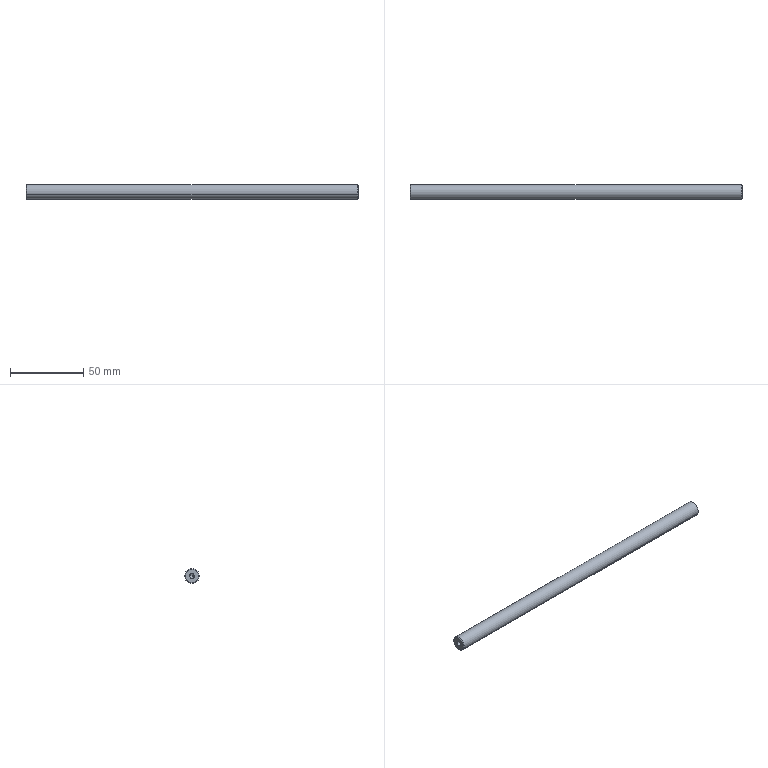Component | SolidWorks | ZL-11-14SupportRod-1 | 1 solid | 16 faces | box 226 x 10 x 10 mm | volume 17564 mm3 | cone 8 | cylinder 6 | plane 2 | commonest cylinder face diameters 3.3 x4 10 x2
build123d program:
from build123d import *

# Parameters (mm, degrees)
SKETCH1_R      = 5
EXTRUDE1_DEPTH = 113
CHAMFER1_SIZE  = 0.5


with BuildPart() as part:
    # Sketch1 → Extrude1 (new, symmetric)
    with BuildSketch(Plane(origin=(0, 0, 0), x_dir=(0, 0, -1), z_dir=(1, 0, 0))):
        Circle(SKETCH1_R)
    extrude(amount=EXTRUDE1_DEPTH, both=True)

    # Chamfer1
    chamfer1_edges = [part.edges().sort_by_distance(p)[0] for p in [
        (-113, 0, 5),
        (113, 0, 5),
    ]]
    chamfer(chamfer1_edges, length=CHAMFER1_SIZE)

    # Sketch2 → M4 Tapped Hole1 (revolve, cut)
    with BuildSketch(Plane(origin=(113, 0, 0), x_dir=(0, 0, -1), z_dir=(0, 1, 0))):
        Polygon((0, 0), (0, 11.091), (1.65, 10.1), (1.65, 0), align=None)
    m4_tapped_hole1 = revolve(axis=Axis((119.35, 0, 0), (-1, 0, 0)), mode=Mode.SUBTRACT)

    # Mirror1: M4 Tapped Hole1 across plane
    add(m4_tapped_hole1.mirror(Plane(origin=(0, 0, 0), x_dir=(0, 0, 1), z_dir=(1, 0, 0))), mode=Mode.SUBTRACT)


solid = part.part

# Placed as in the assembly
solid = solid.moved(Location((-55.448, 283.22, -56), (0, 0, 0)))
STEP:
#1=COLOUR_RGB('',0.7922,0.8196,0.9333);
#2=FILL_AREA_STYLE_COLOUR('',#1);
#3=FILL_AREA_STYLE('',(#2));
#4=SURFACE_STYLE_FILL_AREA(#3);
#5=SURFACE_SIDE_STYLE('',(#4));
#6=SURFACE_STYLE_USAGE(.BOTH.,#5);
#7=PRESENTATION_STYLE_ASSIGNMENT((#6));
#8=CARTESIAN_POINT('',(-6.195,11.15,-2.205));
#9=VERTEX_POINT('',#8);
#10=CARTESIAN_POINT('',(-6.234,11.09,-2.228));
#11=VERTEX_POINT('',#10);
#12=CARTESIAN_POINT('',(-6.234,11.09,-2.228));
#13=DIRECTION('',(-0.515,-0.8026,-0.3009));
#14=VECTOR('',#13,39.37);
#15=LINE('',#12,#14);
#16=EDGE_CURVE('',#9,#11,#15,.T.);
#17=ORIENTED_EDGE('',*,*,#16,.F.);
#18=CARTESIAN_POINT('',(-6.234,11.211,-2.182));
#19=VERTEX_POINT('',#18);
#20=CARTESIAN_POINT('',(-6.234,11.211,-2.182));
#21=DIRECTION('',(-0.515,0.8026,0.3009));
#22=VECTOR('',#21,39.37);
#23=LINE('',#20,#22);
#24=EDGE_CURVE('',#9,#19,#23,.T.);
#25=ORIENTED_EDGE('',*,*,#24,.T.);
#26=CARTESIAN_POINT('',(-6.234,11.15,-2.205));
#27=DIRECTION('',(-1.,0.,0.));
#28=DIRECTION('',(0.,-0.9364,-0.351));
#29=AXIS2_PLACEMENT_3D('',#26,#27,#28);
#30=CIRCLE('',#29,0.06496);
#31=EDGE_CURVE('',#19,#11,#30,.T.);
#32=ORIENTED_EDGE('',*,*,#31,.T.);
#33=EDGE_LOOP('',(#17,#25,#32));
#34=FACE_OUTER_BOUND('',#33,.T.);
#35=CARTESIAN_POINT('',(-6.234,11.15,-2.205));
#36=DIRECTION('',(-1.,0.,0.));
#37=DIRECTION('',(0.,-0.9364,-0.351));
#38=AXIS2_PLACEMENT_3D('',#35,#36,#37);
#39=CONICAL_SURFACE('',#38,0.06496,1.03);
#40=ADVANCED_FACE('',(#34),#39,.F.);
#41=ORIENTED_EDGE('',*,*,#31,.F.);
#42=CARTESIAN_POINT('',(-6.632,11.211,-2.182));
#43=VERTEX_POINT('',#42);
#44=CARTESIAN_POINT('',(-6.632,11.211,-2.182));
#45=DIRECTION('',(-1.,0.,0.));
#46=VECTOR('',#45,39.37);
#47=LINE('',#44,#46);
#48=EDGE_CURVE('',#19,#43,#47,.T.);
#49=ORIENTED_EDGE('',*,*,#48,.T.);
#50=CARTESIAN_POINT('',(-6.632,11.09,-2.228));
#51=VERTEX_POINT('',#50);
#52=CARTESIAN_POINT('',(-6.632,11.15,-2.205));
#53=DIRECTION('',(-1.,0.,0.));
#54=DIRECTION('',(0.,-0.9364,-0.351));
#55=AXIS2_PLACEMENT_3D('',#52,#53,#54);
#56=CIRCLE('',#55,0.06496);
#57=EDGE_CURVE('',#43,#51,#56,.T.);
#58=ORIENTED_EDGE('',*,*,#57,.T.);
#59=CARTESIAN_POINT('',(-6.632,11.09,-2.228));
#60=DIRECTION('',(-1.,0.,0.));
#61=VECTOR('',#60,39.37);
#62=LINE('',#59,#61);
#63=EDGE_CURVE('',#11,#51,#62,.T.);
#64=ORIENTED_EDGE('',*,*,#63,.F.);
#65=EDGE_LOOP('',(#41,#49,#58,#64));
#66=FACE_OUTER_BOUND('',#65,.T.);
#67=CARTESIAN_POINT('',(-6.632,11.15,-2.205));
#68=DIRECTION('',(-1.,0.,0.));
#69=DIRECTION('',(0.,-0.9364,-0.351));
#70=AXIS2_PLACEMENT_3D('',#67,#68,#69);
#71=CYLINDRICAL_SURFACE('',#70,0.06496);
#72=ADVANCED_FACE('',(#66),#71,.F.);
#73=CARTESIAN_POINT('',(1.829,11.15,-2.205));
#74=VERTEX_POINT('',#73);
#75=CARTESIAN_POINT('',(1.868,11.211,-2.182));
#76=VERTEX_POINT('',#75);
#77=CARTESIAN_POINT('',(1.868,11.211,-2.182));
#78=DIRECTION('',(0.515,0.8026,0.3009));
#79=VECTOR('',#78,39.37);
#80=LINE('',#77,#79);
#81=EDGE_CURVE('',#74,#76,#80,.T.);
#82=ORIENTED_EDGE('',*,*,#81,.F.);
#83=CARTESIAN_POINT('',(1.868,11.09,-2.228));
#84=VERTEX_POINT('',#83);
#85=CARTESIAN_POINT('',(1.868,11.09,-2.228));
#86=DIRECTION('',(0.515,-0.8026,-0.3009));
#87=VECTOR('',#86,39.37);
#88=LINE('',#85,#87);
#89=EDGE_CURVE('',#74,#84,#88,.T.);
#90=ORIENTED_EDGE('',*,*,#89,.T.);
#91=CARTESIAN_POINT('',(1.868,11.15,-2.205));
#92=DIRECTION('',(1.,0.,0.));
#93=DIRECTION('',(0.,0.9364,0.351));
#94=AXIS2_PLACEMENT_3D('',#91,#92,#93);
#95=CIRCLE('',#94,0.06496);
#96=EDGE_CURVE('',#84,#76,#95,.T.);
#97=ORIENTED_EDGE('',*,*,#96,.T.);
#98=EDGE_LOOP('',(#82,#90,#97));
#99=FACE_OUTER_BOUND('',#98,.T.);
#100=CARTESIAN_POINT('',(1.868,11.15,-2.205));
#101=DIRECTION('',(1.,0.,0.));
#102=DIRECTION('',(0.,0.9364,0.351));
#103=AXIS2_PLACEMENT_3D('',#100,#101,#102);
#104=CONICAL_SURFACE('',#103,0.06496,1.03);
#105=ADVANCED_FACE('',(#99),#104,.F.);
#106=ORIENTED_EDGE('',*,*,#96,.F.);
#107=CARTESIAN_POINT('',(2.266,11.09,-2.228));
#108=VERTEX_POINT('',#107);
#109=CARTESIAN_POINT('',(2.266,11.09,-2.228));
#110=DIRECTION('',(1.,0.,0.));
#111=VECTOR('',#110,39.37);
#112=LINE('',#109,#111);
#113=EDGE_CURVE('',#84,#108,#112,.T.);
#114=ORIENTED_EDGE('',*,*,#113,.T.);
#115=CARTESIAN_POINT('',(2.266,11.211,-2.182));
#116=VERTEX_POINT('',#115);
#117=CARTESIAN_POINT('',(2.266,11.15,-2.205));
#118=DIRECTION('',(1.,0.,0.));
#119=DIRECTION('',(0.,0.9364,0.351));
#120=AXIS2_PLACEMENT_3D('',#117,#118,#119);
#121=CIRCLE('',#120,0.06496);
#122=EDGE_CURVE('',#108,#116,#121,.T.);
#123=ORIENTED_EDGE('',*,*,#122,.T.);
#124=CARTESIAN_POINT('',(2.266,11.211,-2.182));
#125=DIRECTION('',(1.,0.,0.));
#126=VECTOR('',#125,39.37);
#127=LINE('',#124,#126);
#128=EDGE_CURVE('',#76,#116,#127,.T.);
#129=ORIENTED_EDGE('',*,*,#128,.F.);
#130=EDGE_LOOP('',(#106,#114,#123,#129));
#131=FACE_OUTER_BOUND('',#130,.T.);
#132=CARTESIAN_POINT('',(2.266,11.15,-2.205));
#133=DIRECTION('',(1.,0.,0.));
#134=DIRECTION('',(0.,0.9364,0.351));
#135=AXIS2_PLACEMENT_3D('',#132,#133,#134);
#136=CYLINDRICAL_SURFACE('',#135,0.06496);
#137=ADVANCED_FACE('',(#131),#136,.F.);
#138=CARTESIAN_POINT('',(-6.632,10.984,-2.267));
#139=VERTEX_POINT('',#138);
#140=CARTESIAN_POINT('',(-6.632,11.316,-2.143));
#141=VERTEX_POINT('',#140);
#142=CARTESIAN_POINT('',(-6.632,11.15,-2.205));
#143=DIRECTION('',(-1.,0.,0.));
#144=DIRECTION('',(0.,0.9364,0.351));
#145=AXIS2_PLACEMENT_3D('',#142,#143,#144);
#146=CIRCLE('',#145,0.1772);
#147=EDGE_CURVE('',#139,#141,#146,.T.);
#148=ORIENTED_EDGE('',*,*,#147,.F.);
#149=CARTESIAN_POINT('',(-6.612,10.966,-2.274));
#150=VERTEX_POINT('',#149);
#151=CARTESIAN_POINT('',(-6.612,10.966,-2.274));
#152=DIRECTION('',(0.7071,-0.6621,-0.2482));
#153=VECTOR('',#152,39.37);
#154=LINE('',#151,#153);
#155=EDGE_CURVE('',#139,#150,#154,.T.);
#156=ORIENTED_EDGE('',*,*,#155,.T.);
#157=CARTESIAN_POINT('',(-6.612,11.335,-2.136));
#158=VERTEX_POINT('',#157);
#159=CARTESIAN_POINT('',(-6.612,11.15,-2.205));
#160=DIRECTION('',(1.,0.,0.));
#161=DIRECTION('',(0.,0.9364,0.351));
#162=AXIS2_PLACEMENT_3D('',#159,#160,#161);
#163=CIRCLE('',#162,0.1969);
#164=EDGE_CURVE('',#158,#150,#163,.T.);
#165=ORIENTED_EDGE('',*,*,#164,.F.);
#166=CARTESIAN_POINT('',(-6.612,11.335,-2.136));
#167=DIRECTION('',(0.7071,0.6621,0.2482));
#168=VECTOR('',#167,39.37);
#169=LINE('',#166,#168);
#170=EDGE_CURVE('',#141,#158,#169,.T.);
#171=ORIENTED_EDGE('',*,*,#170,.F.);
#172=EDGE_LOOP('',(#148,#156,#165,#171));
#173=FACE_OUTER_BOUND('',#172,.T.);
#174=CARTESIAN_POINT('',(-6.612,11.15,-2.205));
#175=DIRECTION('',(1.,0.,0.));
#176=DIRECTION('',(0.,0.9364,0.351));
#177=AXIS2_PLACEMENT_3D('',#174,#175,#176);
#178=CONICAL_SURFACE('',#177,0.1969,0.7854);
#179=ADVANCED_FACE('',(#173),#178,.T.);
#180=CARTESIAN_POINT('',(2.266,11.316,-2.143));
#181=VERTEX_POINT('',#180);
#182=CARTESIAN_POINT('',(2.266,10.984,-2.267));
#183=VERTEX_POINT('',#182);
#184=CARTESIAN_POINT('',(2.266,11.15,-2.205));
#185=DIRECTION('',(1.,0.,0.));
#186=DIRECTION('',(0.,0.9364,0.351));
#187=AXIS2_PLACEMENT_3D('',#184,#185,#186);
#188=CIRCLE('',#187,0.1772);
#189=EDGE_CURVE('',#181,#183,#188,.T.);
#190=ORIENTED_EDGE('',*,*,#189,.F.);
#191=CARTESIAN_POINT('',(2.246,11.335,-2.136));
#192=VERTEX_POINT('',#191);
#193=CARTESIAN_POINT('',(2.266,11.316,-2.143));
#194=DIRECTION('',(-0.7071,0.6621,0.2482));
#195=VECTOR('',#194,39.37);
#196=LINE('',#193,#195);
#197=EDGE_CURVE('',#181,#192,#196,.T.);
#198=ORIENTED_EDGE('',*,*,#197,.T.);
#199=CARTESIAN_POINT('',(2.246,10.966,-2.274));
#200=VERTEX_POINT('',#199);
#201=CARTESIAN_POINT('',(2.246,11.15,-2.205));
#202=DIRECTION('',(-1.,0.,0.));
#203=DIRECTION('',(0.,0.9364,0.351));
#204=AXIS2_PLACEMENT_3D('',#201,#202,#203);
#205=CIRCLE('',#204,0.1969);
#206=EDGE_CURVE('',#200,#192,#205,.T.);
#207=ORIENTED_EDGE('',*,*,#206,.F.);
#208=CARTESIAN_POINT('',(2.266,10.984,-2.267));
#209=DIRECTION('',(-0.7071,-0.6621,-0.2482));
#210=VECTOR('',#209,39.37);
#211=LINE('',#208,#210);
#212=EDGE_CURVE('',#183,#200,#211,.T.);
#213=ORIENTED_EDGE('',*,*,#212,.F.);
#214=EDGE_LOOP('',(#190,#198,#207,#213));
#215=FACE_OUTER_BOUND('',#214,.T.);
#216=CARTESIAN_POINT('',(2.266,11.15,-2.205));
#217=DIRECTION('',(-1.,0.,0.));
#218=DIRECTION('',(0.,-0.9364,-0.351));
#219=AXIS2_PLACEMENT_3D('',#216,#217,#218);
#220=CONICAL_SURFACE('',#219,0.1772,0.7854);
#221=ADVANCED_FACE('',(#215),#220,.T.);
#222=ORIENTED_EDGE('',*,*,#206,.T.);
#223=CARTESIAN_POINT('',(2.266,11.335,-2.136));
#224=DIRECTION('',(-1.,0.,0.));
#225=VECTOR('',#224,39.37);
#226=LINE('',#223,#225);
#227=EDGE_CURVE('',#192,#158,#226,.T.);
#228=ORIENTED_EDGE('',*,*,#227,.T.);
#229=ORIENTED_EDGE('',*,*,#164,.T.);
#230=CARTESIAN_POINT('',(2.266,10.966,-2.274));
#231=DIRECTION('',(-1.,0.,0.));
#232=VECTOR('',#231,39.37);
#233=LINE('',#230,#232);
#234=EDGE_CURVE('',#200,#150,#233,.T.);
#235=ORIENTED_EDGE('',*,*,#234,.F.);
#236=EDGE_LOOP('',(#222,#228,#229,#235));
#237=FACE_OUTER_BOUND('',#236,.T.);
#238=CARTESIAN_POINT('',(2.266,11.15,-2.205));
#239=DIRECTION('',(-1.,0.,0.));
#240=DIRECTION('',(0.,-0.9364,-0.351));
#241=AXIS2_PLACEMENT_3D('',#238,#239,#240);
#242=CYLINDRICAL_SURFACE('',#241,0.1969);
#243=ADVANCED_FACE('',(#237),#242,.T.);
#244=ORIENTED_EDGE('',*,*,#227,.F.);
#245=CARTESIAN_POINT('',(2.246,11.15,-2.205));
#246=DIRECTION('',(-1.,0.,0.));
#247=DIRECTION('',(0.,0.9364,0.351));
#248=AXIS2_PLACEMENT_3D('',#245,#246,#247);
#249=CIRCLE('',#248,0.1969);
#250=EDGE_CURVE('',#192,#200,#249,.T.);
#251=ORIENTED_EDGE('',*,*,#250,.T.);
#252=ORIENTED_EDGE('',*,*,#234,.T.);
#253=CARTESIAN_POINT('',(-6.612,11.15,-2.205));
#254=DIRECTION('',(1.,0.,0.));
#255=DIRECTION('',(0.,0.9364,0.351));
#256=AXIS2_PLACEMENT_3D('',#253,#254,#255);
#257=CIRCLE('',#256,0.1969);
#258=EDGE_CURVE('',#150,#158,#257,.T.);
#259=ORIENTED_EDGE('',*,*,#258,.T.);
#260=EDGE_LOOP('',(#244,#251,#252,#259));
#261=FACE_OUTER_BOUND('',#260,.T.);
#262=CARTESIAN_POINT('',(2.266,11.15,-2.205));
#263=DIRECTION('',(-1.,0.,0.));
#264=DIRECTION('',(0.,-0.9364,-0.351));
#265=AXIS2_PLACEMENT_3D('',#262,#263,#264);
#266=CYLINDRICAL_SURFACE('',#265,0.1969);
#267=ADVANCED_FACE('',(#261),#266,.T.);
#268=CARTESIAN_POINT('',(2.266,11.15,-2.205));
#269=DIRECTION('',(1.,0.,0.));
#270=DIRECTION('',(0.,0.9364,0.351));
#271=AXIS2_PLACEMENT_3D('',#268,#269,#270);
#272=CIRCLE('',#271,0.06496);
#273=EDGE_CURVE('',#116,#108,#272,.T.);
#274=ORIENTED_EDGE('',*,*,#273,.F.);
#275=ORIENTED_EDGE('',*,*,#122,.F.);
#276=EDGE_LOOP('',(#274,#275));
#277=FACE_BOUND('',#276,.T.);
#278=CARTESIAN_POINT('',(2.266,11.15,-2.205));
#279=DIRECTION('',(1.,0.,0.));
#280=DIRECTION('',(0.,0.9364,0.351));
#281=AXIS2_PLACEMENT_3D('',#278,#279,#280);
#282=CIRCLE('',#281,0.1772);
#283=EDGE_CURVE('',#183,#181,#282,.T.);
#284=ORIENTED_EDGE('',*,*,#283,.T.);
#285=ORIENTED_EDGE('',*,*,#189,.T.);
#286=EDGE_LOOP('',(#284,#285));
#287=FACE_OUTER_BOUND('',#286,.T.);
#288=CARTESIAN_POINT('',(2.266,11.15,-2.205));
#289=DIRECTION('',(1.,0.,0.));
#290=DIRECTION('',(0.,0.9364,0.351));
#291=AXIS2_PLACEMENT_3D('',#288,#289,#290);
#292=PLANE('',#291);
#293=ADVANCED_FACE('',(#277,#287),#292,.T.);
#294=CARTESIAN_POINT('',(-6.632,11.15,-2.205));
#295=DIRECTION('',(-1.,0.,0.));
#296=DIRECTION('',(0.,-0.9364,-0.351));
#297=AXIS2_PLACEMENT_3D('',#294,#295,#296);
#298=CIRCLE('',#297,0.06496);
#299=EDGE_CURVE('',#51,#43,#298,.T.);
#300=ORIENTED_EDGE('',*,*,#299,.F.);
#301=ORIENTED_EDGE('',*,*,#57,.F.);
#302=EDGE_LOOP('',(#300,#301));
#303=FACE_BOUND('',#302,.T.);
#304=CARTESIAN_POINT('',(-6.632,11.15,-2.205));
#305=DIRECTION('',(-1.,0.,0.));
#306=DIRECTION('',(0.,0.9364,0.351));
#307=AXIS2_PLACEMENT_3D('',#304,#305,#306);
#308=CIRCLE('',#307,0.1772);
#309=EDGE_CURVE('',#141,#139,#308,.T.);
#310=ORIENTED_EDGE('',*,*,#309,.T.);
#311=ORIENTED_EDGE('',*,*,#147,.T.);
#312=EDGE_LOOP('',(#310,#311));
#313=FACE_OUTER_BOUND('',#312,.T.);
#314=CARTESIAN_POINT('',(-6.632,11.15,-2.205));
#315=DIRECTION('',(1.,0.,0.));
#316=DIRECTION('',(0.,0.9364,0.351));
#317=AXIS2_PLACEMENT_3D('',#314,#315,#316);
#318=PLANE('',#317);
#319=ADVANCED_FACE('',(#303,#313),#318,.F.);
#320=ORIENTED_EDGE('',*,*,#197,.F.);
#321=ORIENTED_EDGE('',*,*,#283,.F.);
#322=ORIENTED_EDGE('',*,*,#212,.T.);
#323=ORIENTED_EDGE('',*,*,#250,.F.);
#324=EDGE_LOOP('',(#320,#321,#322,#323));
#325=FACE_OUTER_BOUND('',#324,.T.);
#326=CARTESIAN_POINT('',(2.266,11.15,-2.205));
#327=DIRECTION('',(-1.,0.,0.));
#328=DIRECTION('',(0.,-0.9364,-0.351));
#329=AXIS2_PLACEMENT_3D('',#326,#327,#328);
#330=CONICAL_SURFACE('',#329,0.1772,0.7854);
#331=ADVANCED_FACE('',(#325),#330,.T.);
#332=ORIENTED_EDGE('',*,*,#155,.F.);
#333=ORIENTED_EDGE('',*,*,#309,.F.);
#334=ORIENTED_EDGE('',*,*,#170,.T.);
#335=ORIENTED_EDGE('',*,*,#258,.F.);
#336=EDGE_LOOP('',(#332,#333,#334,#335));
#337=FACE_OUTER_BOUND('',#336,.T.);
#338=CARTESIAN_POINT('',(-6.612,11.15,-2.205));
#339=DIRECTION('',(1.,0.,0.));
#340=DIRECTION('',(0.,0.9364,0.351));
#341=AXIS2_PLACEMENT_3D('',#338,#339,#340);
#342=CONICAL_SURFACE('',#341,0.1969,0.7854);
#343=ADVANCED_FACE('',(#337),#342,.T.);
#344=ORIENTED_EDGE('',*,*,#113,.F.);
#345=CARTESIAN_POINT('',(1.868,11.15,-2.205));
#346=DIRECTION('',(1.,0.,0.));
#347=DIRECTION('',(0.,0.9364,0.351));
#348=AXIS2_PLACEMENT_3D('',#345,#346,#347);
#349=CIRCLE('',#348,0.06496);
#350=EDGE_CURVE('',#76,#84,#349,.T.);
#351=ORIENTED_EDGE('',*,*,#350,.F.);
#352=ORIENTED_EDGE('',*,*,#128,.T.);
#353=ORIENTED_EDGE('',*,*,#273,.T.);
#354=EDGE_LOOP('',(#344,#351,#352,#353));
#355=FACE_OUTER_BOUND('',#354,.T.);
#356=CARTESIAN_POINT('',(2.266,11.15,-2.205));
#357=DIRECTION('',(1.,0.,0.));
#358=DIRECTION('',(0.,0.9364,0.351));
#359=AXIS2_PLACEMENT_3D('',#356,#357,#358);
#360=CYLINDRICAL_SURFACE('',#359,0.06496);
#361=ADVANCED_FACE('',(#355),#360,.F.);
#362=ORIENTED_EDGE('',*,*,#89,.F.);
#363=ORIENTED_EDGE('',*,*,#81,.T.);
#364=ORIENTED_EDGE('',*,*,#350,.T.);
#365=EDGE_LOOP('',(#362,#363,#364));
#366=FACE_OUTER_BOUND('',#365,.T.);
#367=CARTESIAN_POINT('',(1.868,11.15,-2.205));
#368=DIRECTION('',(1.,0.,0.));
#369=DIRECTION('',(0.,0.9364,0.351));
#370=AXIS2_PLACEMENT_3D('',#367,#368,#369);
#371=CONICAL_SURFACE('',#370,0.06496,1.03);
#372=ADVANCED_FACE('',(#366),#371,.F.);
#373=ORIENTED_EDGE('',*,*,#48,.F.);
#374=CARTESIAN_POINT('',(-6.234,11.15,-2.205));
#375=DIRECTION('',(-1.,0.,0.));
#376=DIRECTION('',(0.,-0.9364,-0.351));
#377=AXIS2_PLACEMENT_3D('',#374,#375,#376);
#378=CIRCLE('',#377,0.06496);
#379=EDGE_CURVE('',#11,#19,#378,.T.);
#380=ORIENTED_EDGE('',*,*,#379,.F.);
#381=ORIENTED_EDGE('',*,*,#63,.T.);
#382=ORIENTED_EDGE('',*,*,#299,.T.);
#383=EDGE_LOOP('',(#373,#380,#381,#382));
#384=FACE_OUTER_BOUND('',#383,.T.);
#385=CARTESIAN_POINT('',(-6.632,11.15,-2.205));
#386=DIRECTION('',(-1.,0.,0.));
#387=DIRECTION('',(0.,-0.9364,-0.351));
#388=AXIS2_PLACEMENT_3D('',#385,#386,#387);
#389=CYLINDRICAL_SURFACE('',#388,0.06496);
#390=ADVANCED_FACE('',(#384),#389,.F.);
#391=ORIENTED_EDGE('',*,*,#24,.F.);
#392=ORIENTED_EDGE('',*,*,#16,.T.);
#393=ORIENTED_EDGE('',*,*,#379,.T.);
#394=EDGE_LOOP('',(#391,#392,#393));
#395=FACE_OUTER_BOUND('',#394,.T.);
#396=CARTESIAN_POINT('',(-6.234,11.15,-2.205));
#397=DIRECTION('',(-1.,0.,0.));
#398=DIRECTION('',(0.,-0.9364,-0.351));
#399=AXIS2_PLACEMENT_3D('',#396,#397,#398);
#400=CONICAL_SURFACE('',#399,0.06496,1.03);
#401=ADVANCED_FACE('',(#395),#400,.F.);
#402=CLOSED_SHELL('',(#40,#72,#105,#137,#179,#221,#243,#267,#293,#319,#331,#343,#361,#372,#390,#401));
#403=MANIFOLD_SOLID_BREP('',#402);
#404=STYLED_ITEM('',(#7),#403);
#405=(LENGTH_UNIT()NAMED_UNIT(*)SI_UNIT($,.METRE.));
#406=LENGTH_MEASURE_WITH_UNIT(LENGTH_MEASURE(0.0254),#405);
#407=DIMENSIONAL_EXPONENTS(1.,0.,0.,0.,0.,0.,0.);
#408=(CONVERSION_BASED_UNIT('',#406)LENGTH_UNIT()NAMED_UNIT(#407));
#409=UNCERTAINTY_MEASURE_WITH_UNIT(LENGTH_MEASURE(0.00001),#408,'','');
#410=(NAMED_UNIT(*)PLANE_ANGLE_UNIT()SI_UNIT($,.RADIAN.));
#411=(NAMED_UNIT(*)SI_UNIT($,.STERADIAN.)SOLID_ANGLE_UNIT());
#412=(GEOMETRIC_REPRESENTATION_CONTEXT(3)GLOBAL_UNCERTAINTY_ASSIGNED_CONTEXT((#409))GLOBAL_UNIT_ASSIGNED_CONTEXT((#408,#410,#411))REPRESENTATION_CONTEXT('',''));
#413=MECHANICAL_DESIGN_GEOMETRIC_PRESENTATION_REPRESENTATION('',(#404),#412);
#414=PRESENTATION_LAYER_ASSIGNMENT('','',(#404));
#415=CARTESIAN_POINT('',(0.,0.,0.));
#416=DIRECTION('',(0.,0.,1.));
#417=DIRECTION('',(1.,0.,0.));
#418=AXIS2_PLACEMENT_3D('',#415,#416,#417);
#419=(LENGTH_UNIT()NAMED_UNIT(*)SI_UNIT($,.METRE.));
#420=LENGTH_MEASURE_WITH_UNIT(LENGTH_MEASURE(0.0254),#419);
#421=DIMENSIONAL_EXPONENTS(1.,0.,0.,0.,0.,0.,0.);
#422=(CONVERSION_BASED_UNIT('',#420)LENGTH_UNIT()NAMED_UNIT(#421));
#423=UNCERTAINTY_MEASURE_WITH_UNIT(LENGTH_MEASURE(0.00001),#422,'','');
#424=(NAMED_UNIT(*)PLANE_ANGLE_UNIT()SI_UNIT($,.RADIAN.));
#425=(NAMED_UNIT(*)SI_UNIT($,.STERADIAN.)SOLID_ANGLE_UNIT());
#426=(GEOMETRIC_REPRESENTATION_CONTEXT(3)GLOBAL_UNCERTAINTY_ASSIGNED_CONTEXT((#423))GLOBAL_UNIT_ASSIGNED_CONTEXT((#422,#424,#425))REPRESENTATION_CONTEXT('',''));
#427=ADVANCED_BREP_SHAPE_REPRESENTATION('',(#403,#418),#426);